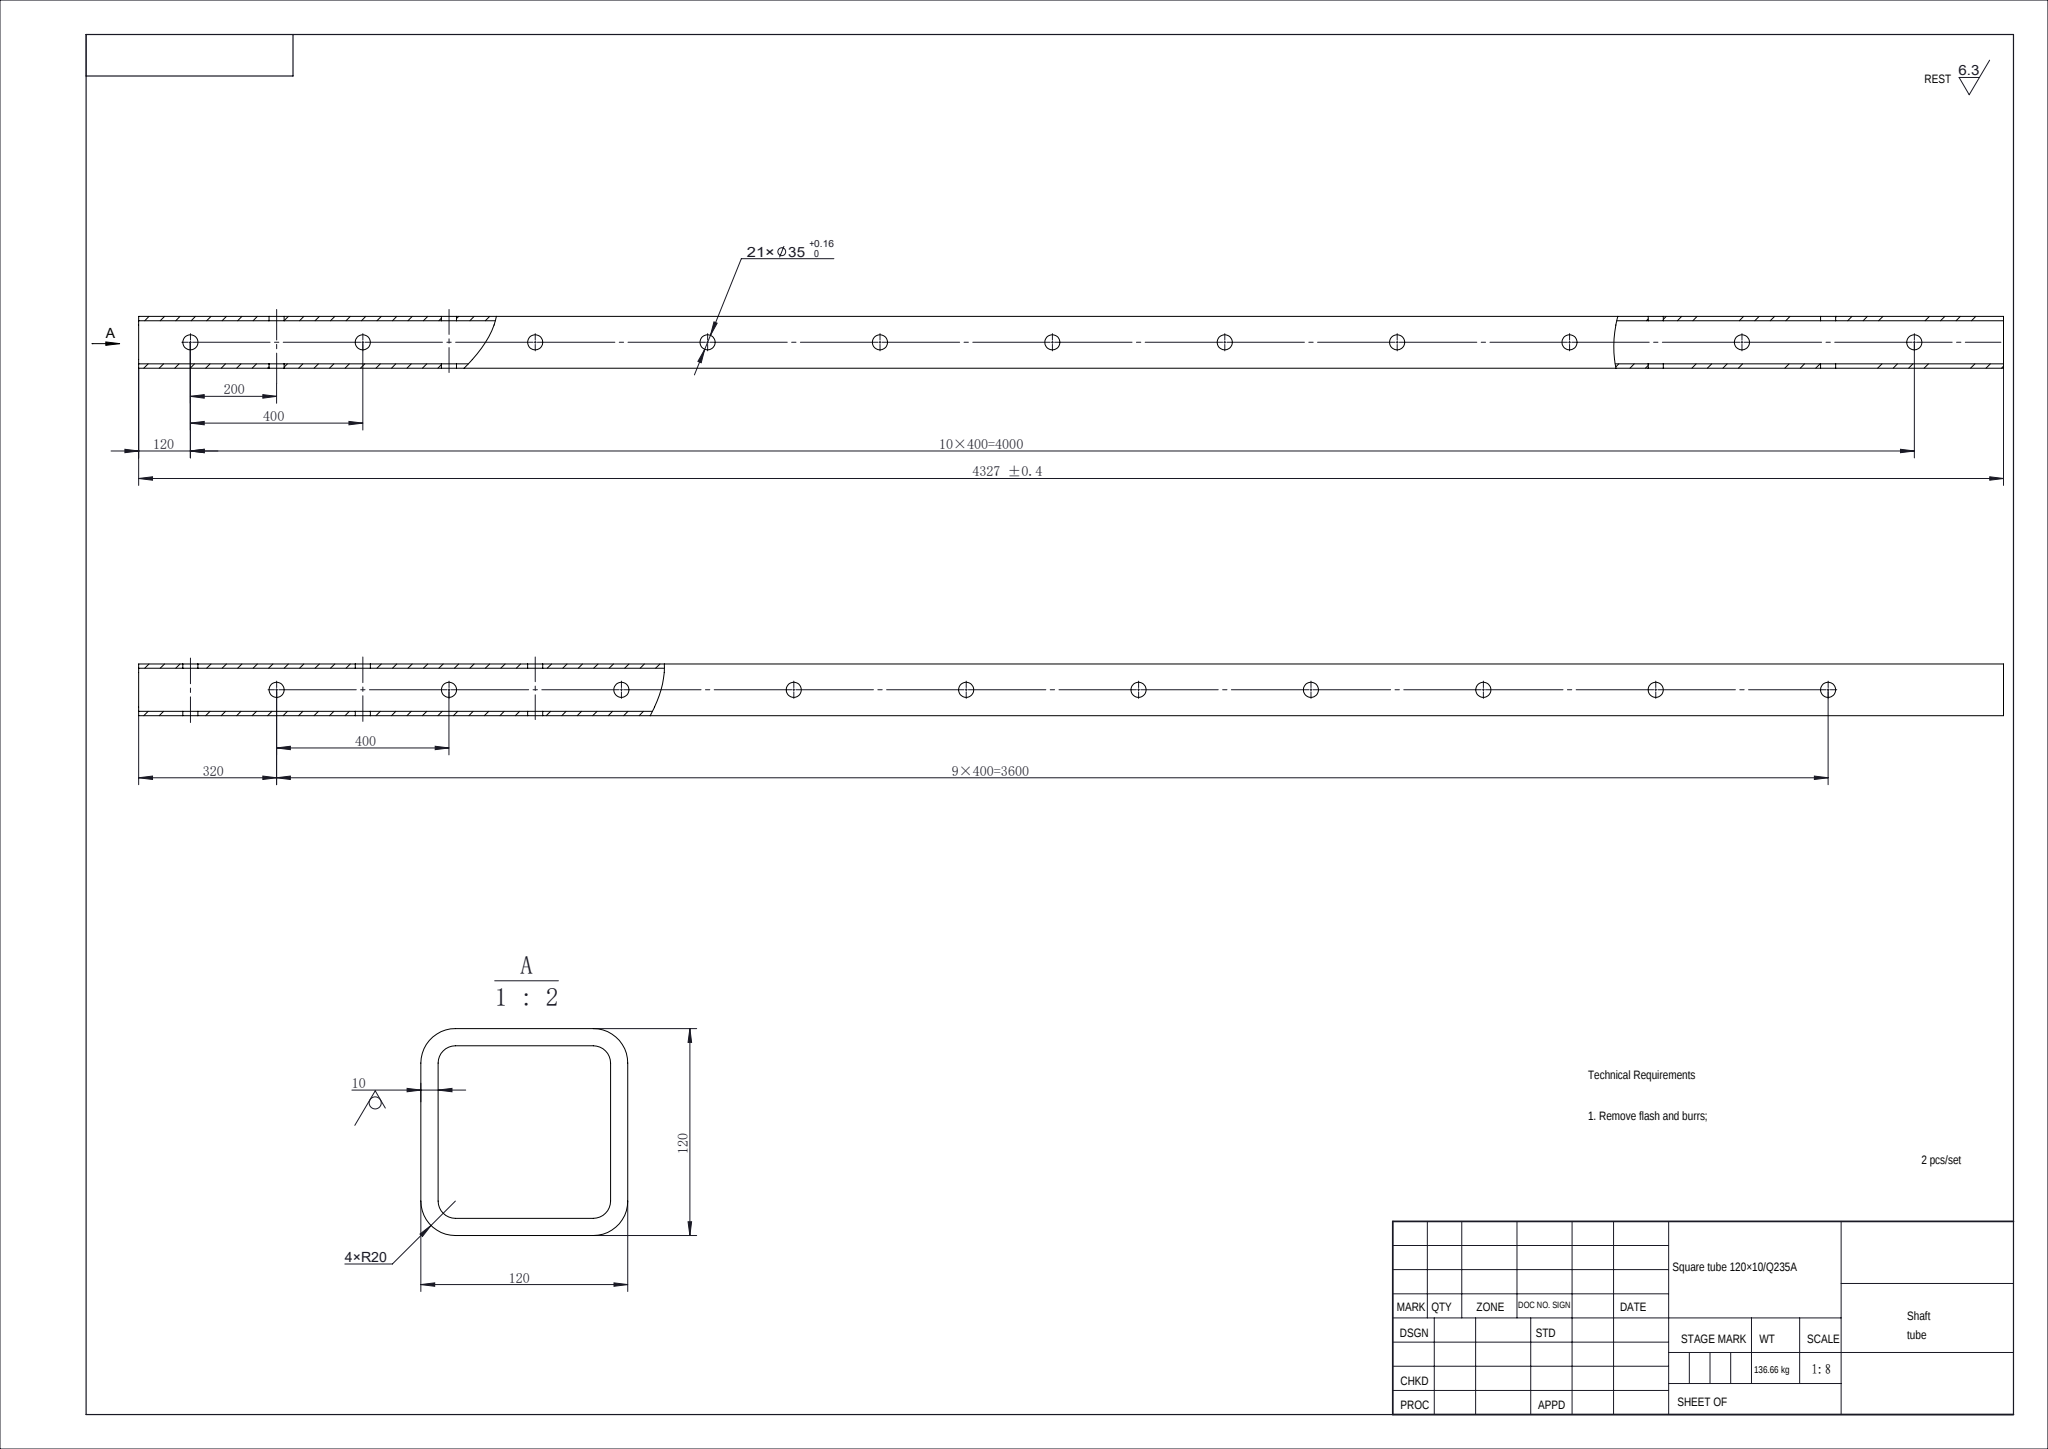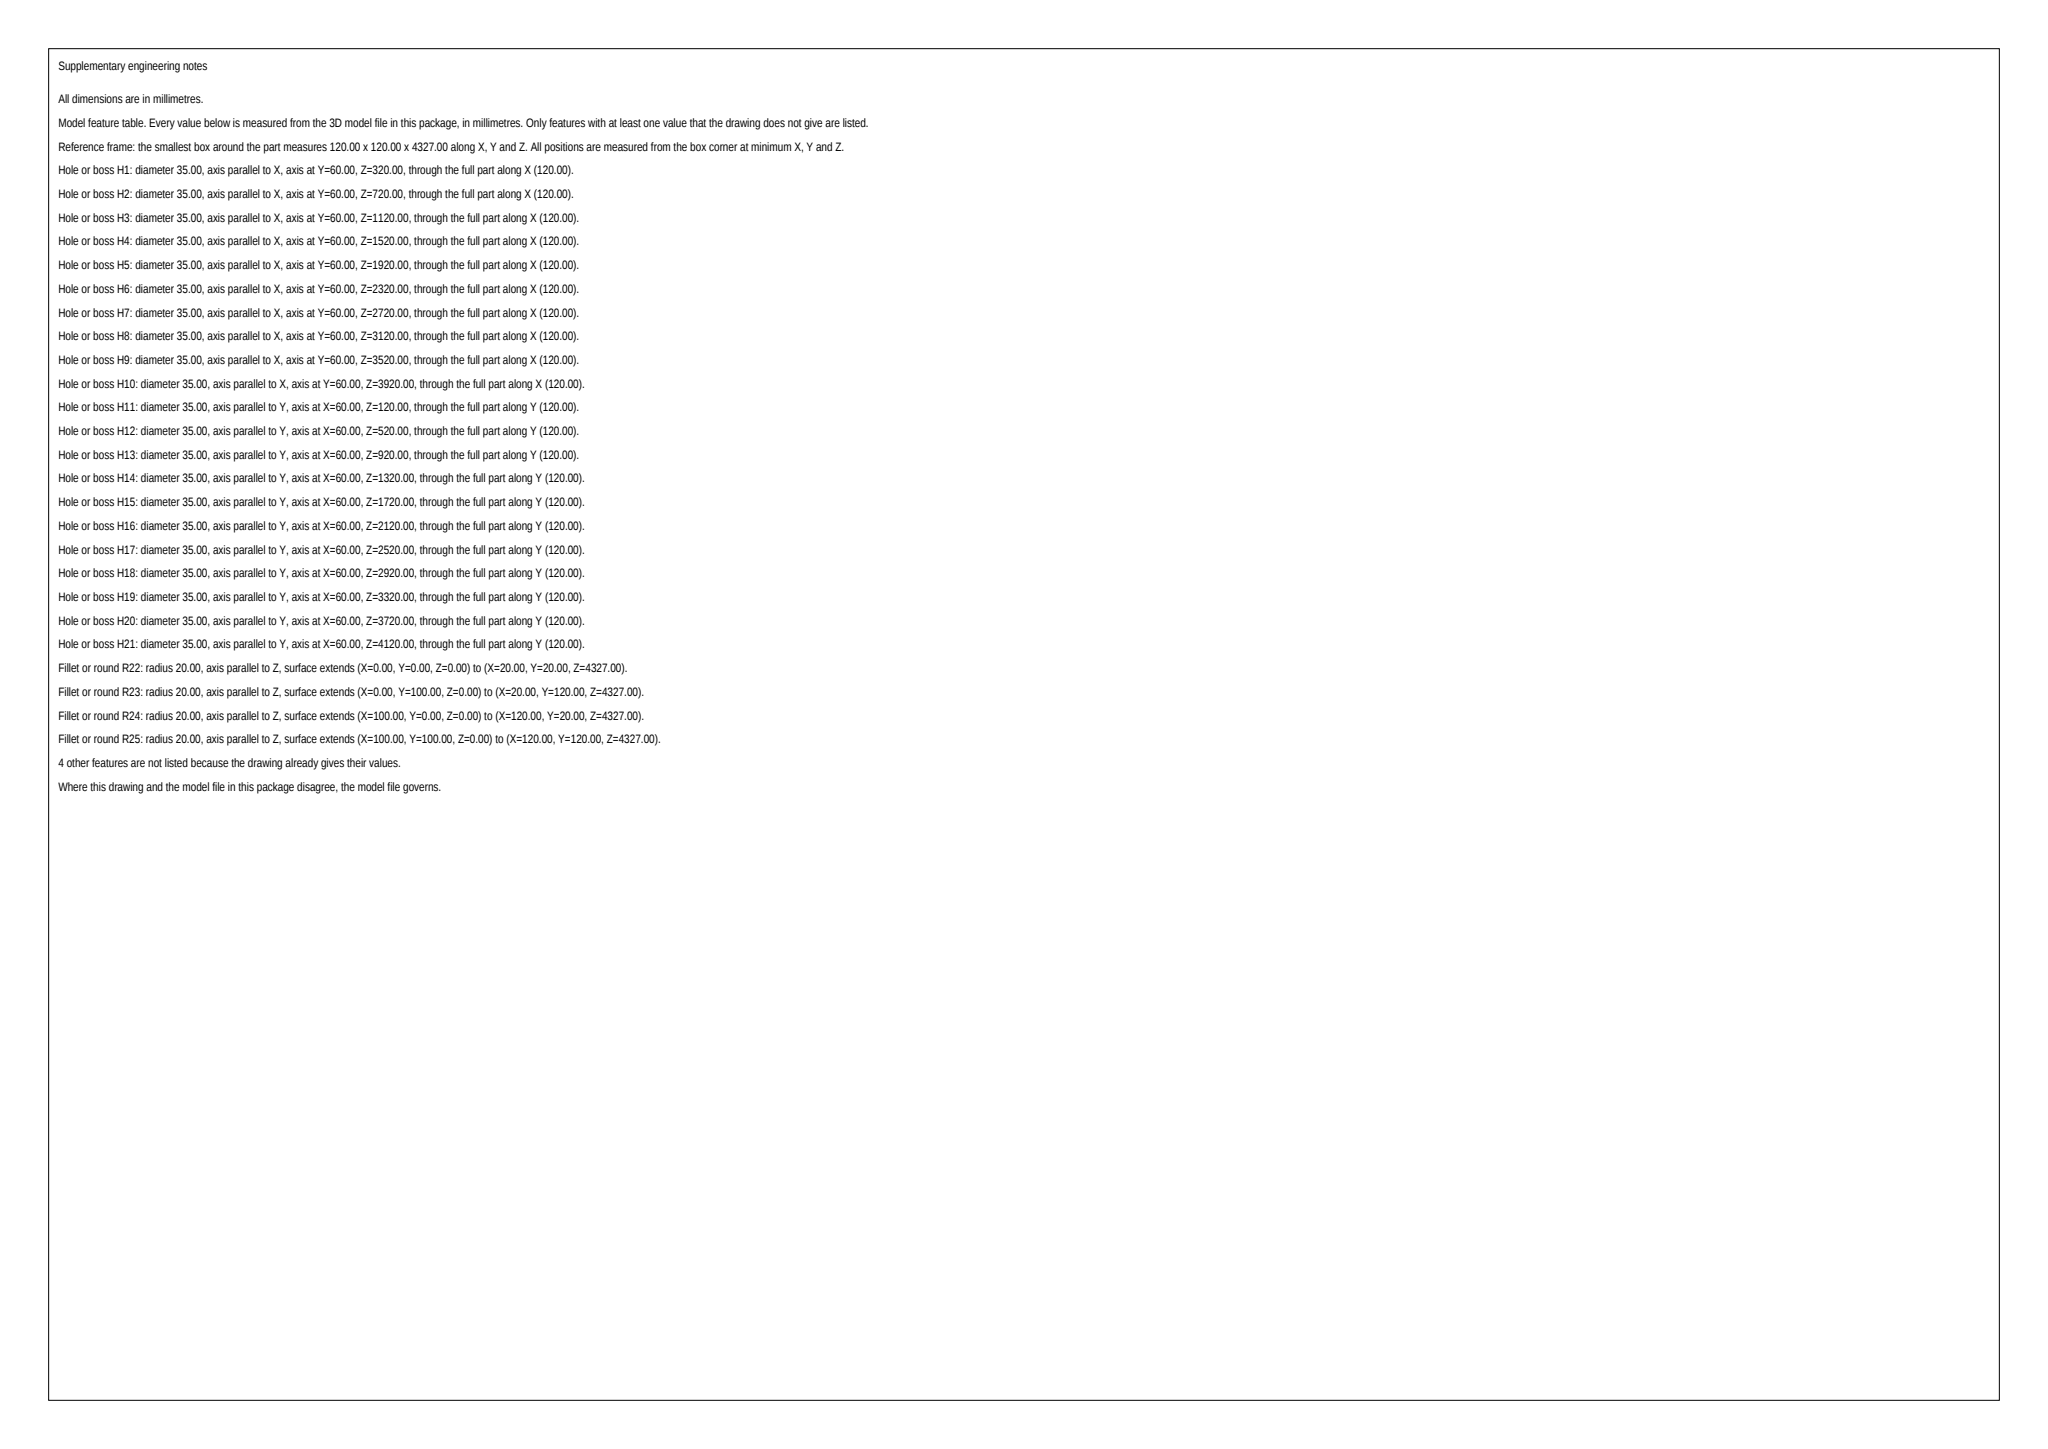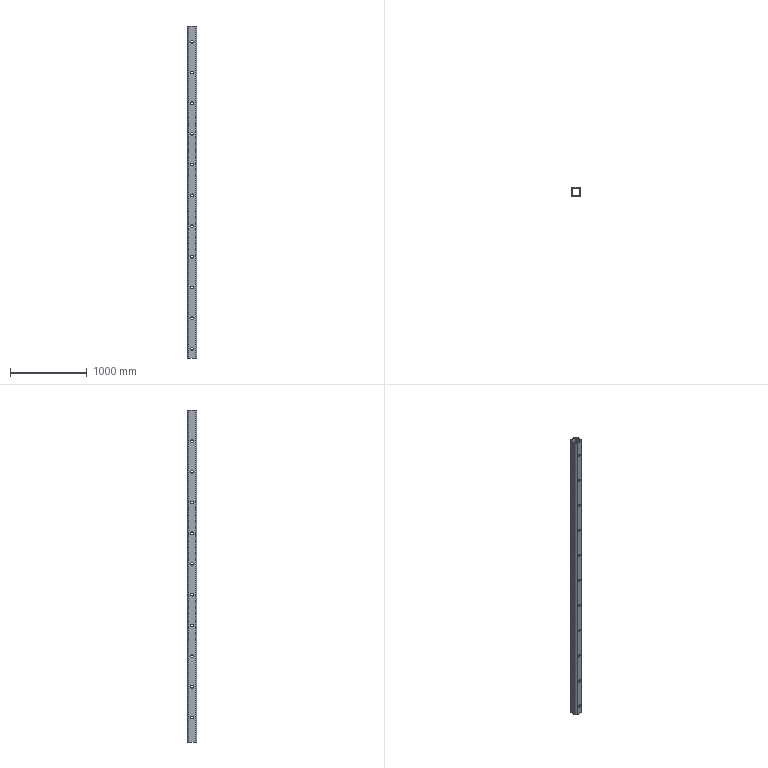Part | SolidWorks | mm | material Square tube 120×10/Q235A | 1 solid | 102 faces | box 120 x 120 x 4327 mm | volume 17520414 mm3 | cylinder 92 | plane 10 | commonest cylinder face diameters 35 x84 20 x4 40 x4
build123d program:
from build123d import *

# Parameters (mm, degrees)
SKETCH1_W               = 120
SKETCH1_H               = 120
SKETCH1_W_2             = 100
SKETCH1_H_2             = 100
BOSS_EXTRUDE1_DEPTH     = 4327
CUT_EXTRUDE3_DEPTH      = 4328.832
CUT_EXTRUDE3_DEPTH_BACK = 4328.832
SKETCH4_R               = 17.5
CUT_EXTRUDE4_DEPTH      = 4328.832
CUT_EXTRUDE4_DEPTH_BACK = 4328.832
SKETCH5_R               = 17.5
FILLET1_R               = 10
FILLET2_R               = 20


with BuildPart() as part:
    # Sketch1 → Boss-Extrude1 (new body)
    with BuildSketch(Plane.XY):
        Rectangle(SKETCH1_W, SKETCH1_H)
        Rectangle(SKETCH1_W_2, SKETCH1_H_2, mode=Mode.SUBTRACT)
    extrude(amount=BOSS_EXTRUDE1_DEPTH)

    # Sketch4 → Cut-Extrude3 (cut, two sides: drawn at the far end of the back side and taken through both)
    with BuildSketch(Plane(origin=(0, 0, 0), x_dir=(1, 0, 0), z_dir=(0, 1, 0)).offset(-CUT_EXTRUDE3_DEPTH_BACK)):
        with Locations(Location((0, -120, 0), (0, 0, 270))):
            Circle(SKETCH4_R)
        with Locations(Location((0, -520, 0), (0, 0, 270))):
            Circle(SKETCH4_R)
        with Locations(Location((0, -920, 0), (0, 0, 270))):
            Circle(SKETCH4_R)
        with Locations(Location((0, -1320, 0), (0, 0, 270))):
            Circle(SKETCH4_R)
        with Locations(Location((0, -1720, 0), (0, 0, 270))):
            Circle(SKETCH4_R)
        with Locations(Location((0, -2120, 0), (0, 0, 270))):
            Circle(SKETCH4_R)
        with Locations(Location((0, -2520, 0), (0, 0, 270))):
            Circle(SKETCH4_R)
        with Locations(Location((0, -2920, 0), (0, 0, 270))):
            Circle(SKETCH4_R)
        with Locations(Location((0, -3320, 0), (0, 0, 270))):
            Circle(SKETCH4_R)
        with Locations(Location((0, -3720, 0), (0, 0, 270))):
            Circle(SKETCH4_R)
        with Locations(Location((0, -4120, 0), (0, 0, 270))):
            Circle(SKETCH4_R)
    extrude(amount=CUT_EXTRUDE3_DEPTH + CUT_EXTRUDE3_DEPTH_BACK, mode=Mode.SUBTRACT)

    # Sketch5 → Cut-Extrude4 (cut, two sides: drawn at the far end of the back side and taken through both)
    with BuildSketch(Plane(origin=(0, 0, 0), x_dir=(0, 0, -1), z_dir=(1, 0, 0)).offset(-CUT_EXTRUDE4_DEPTH_BACK)):
        with Locations((-320, 0)):
            Circle(SKETCH5_R)
        with Locations((-720, 0)):
            Circle(SKETCH5_R)
        with Locations((-1120, 0)):
            Circle(SKETCH5_R)
        with Locations((-1520, 0)):
            Circle(SKETCH5_R)
        with Locations((-1920, 0)):
            Circle(SKETCH5_R)
        with Locations((-2320, 0)):
            Circle(SKETCH5_R)
        with Locations((-2720, 0)):
            Circle(SKETCH5_R)
        with Locations((-3120, 0)):
            Circle(SKETCH5_R)
        with Locations((-3520, 0)):
            Circle(SKETCH5_R)
        with Locations((-3920, 0)):
            Circle(SKETCH5_R)
    extrude(amount=CUT_EXTRUDE4_DEPTH + CUT_EXTRUDE4_DEPTH_BACK, mode=Mode.SUBTRACT)

    # Fillet1
    fillet1_edges = [part.edges().sort_by_distance(p)[0] for p in [
        (50, -50, 2163.5),
        (50, 50, 2163.5),
        (-50, 50, 2163.5),
        (-50, -50, 2163.5),
    ]]
    fillet(fillet1_edges, radius=FILLET1_R)

    # Fillet2
    fillet2_edges = [part.edges().sort_by_distance(p)[0] for p in [
        (60, -60, 2163.5),
        (-60, -60, 2163.5),
        (-60, 60, 2163.5),
        (60, 60, 2163.5),
    ]]
    fillet(fillet2_edges, radius=FILLET2_R)


solid = part.part